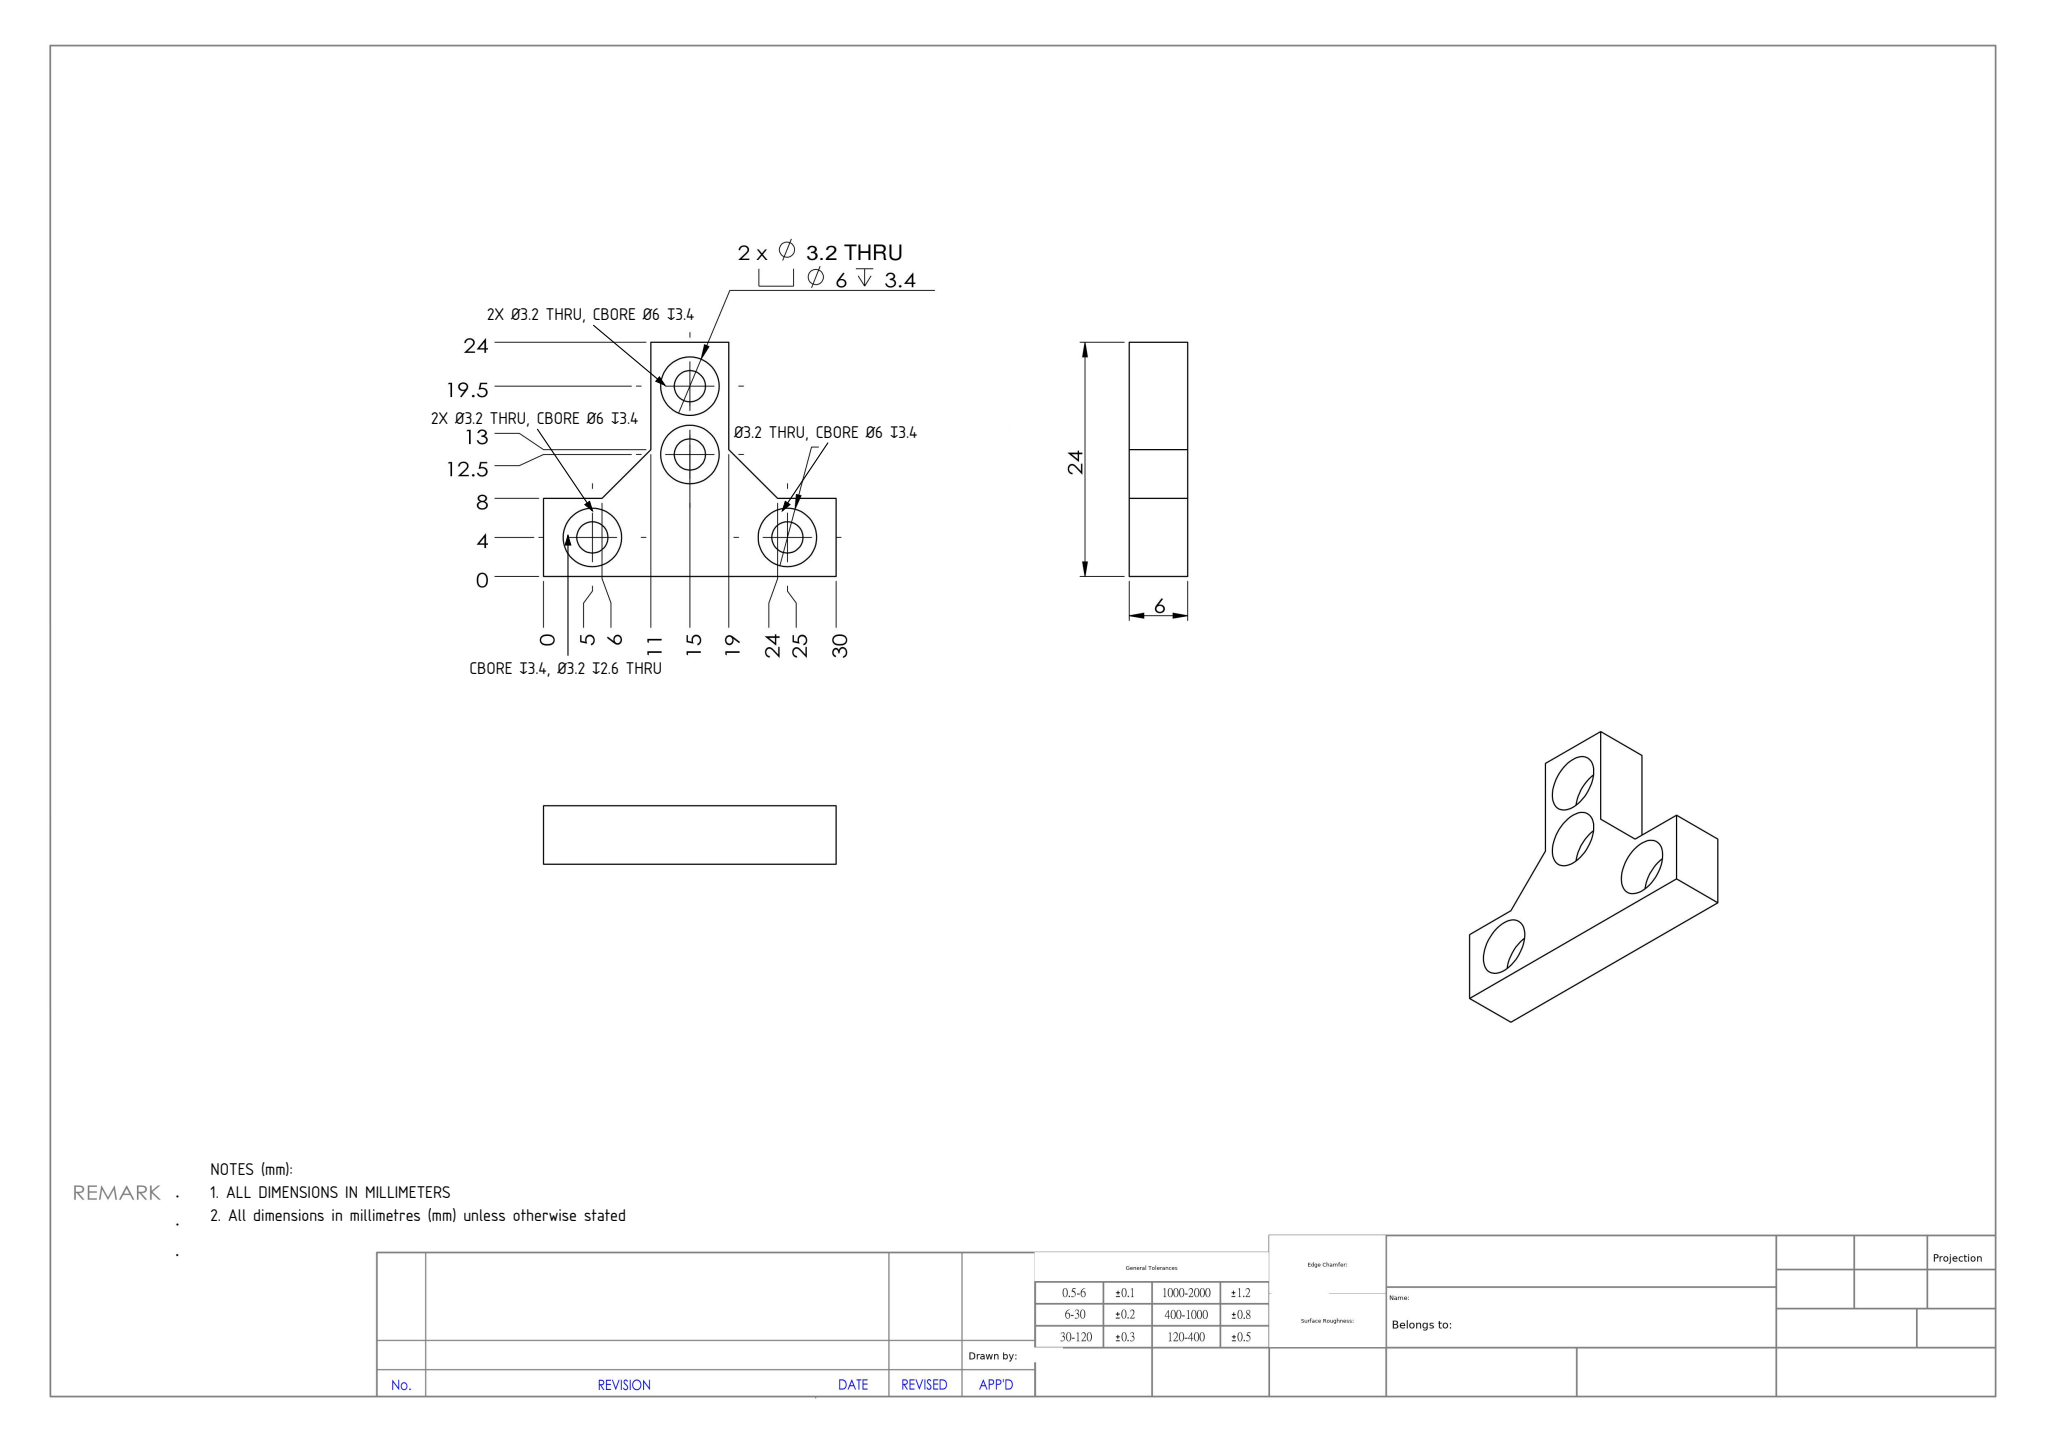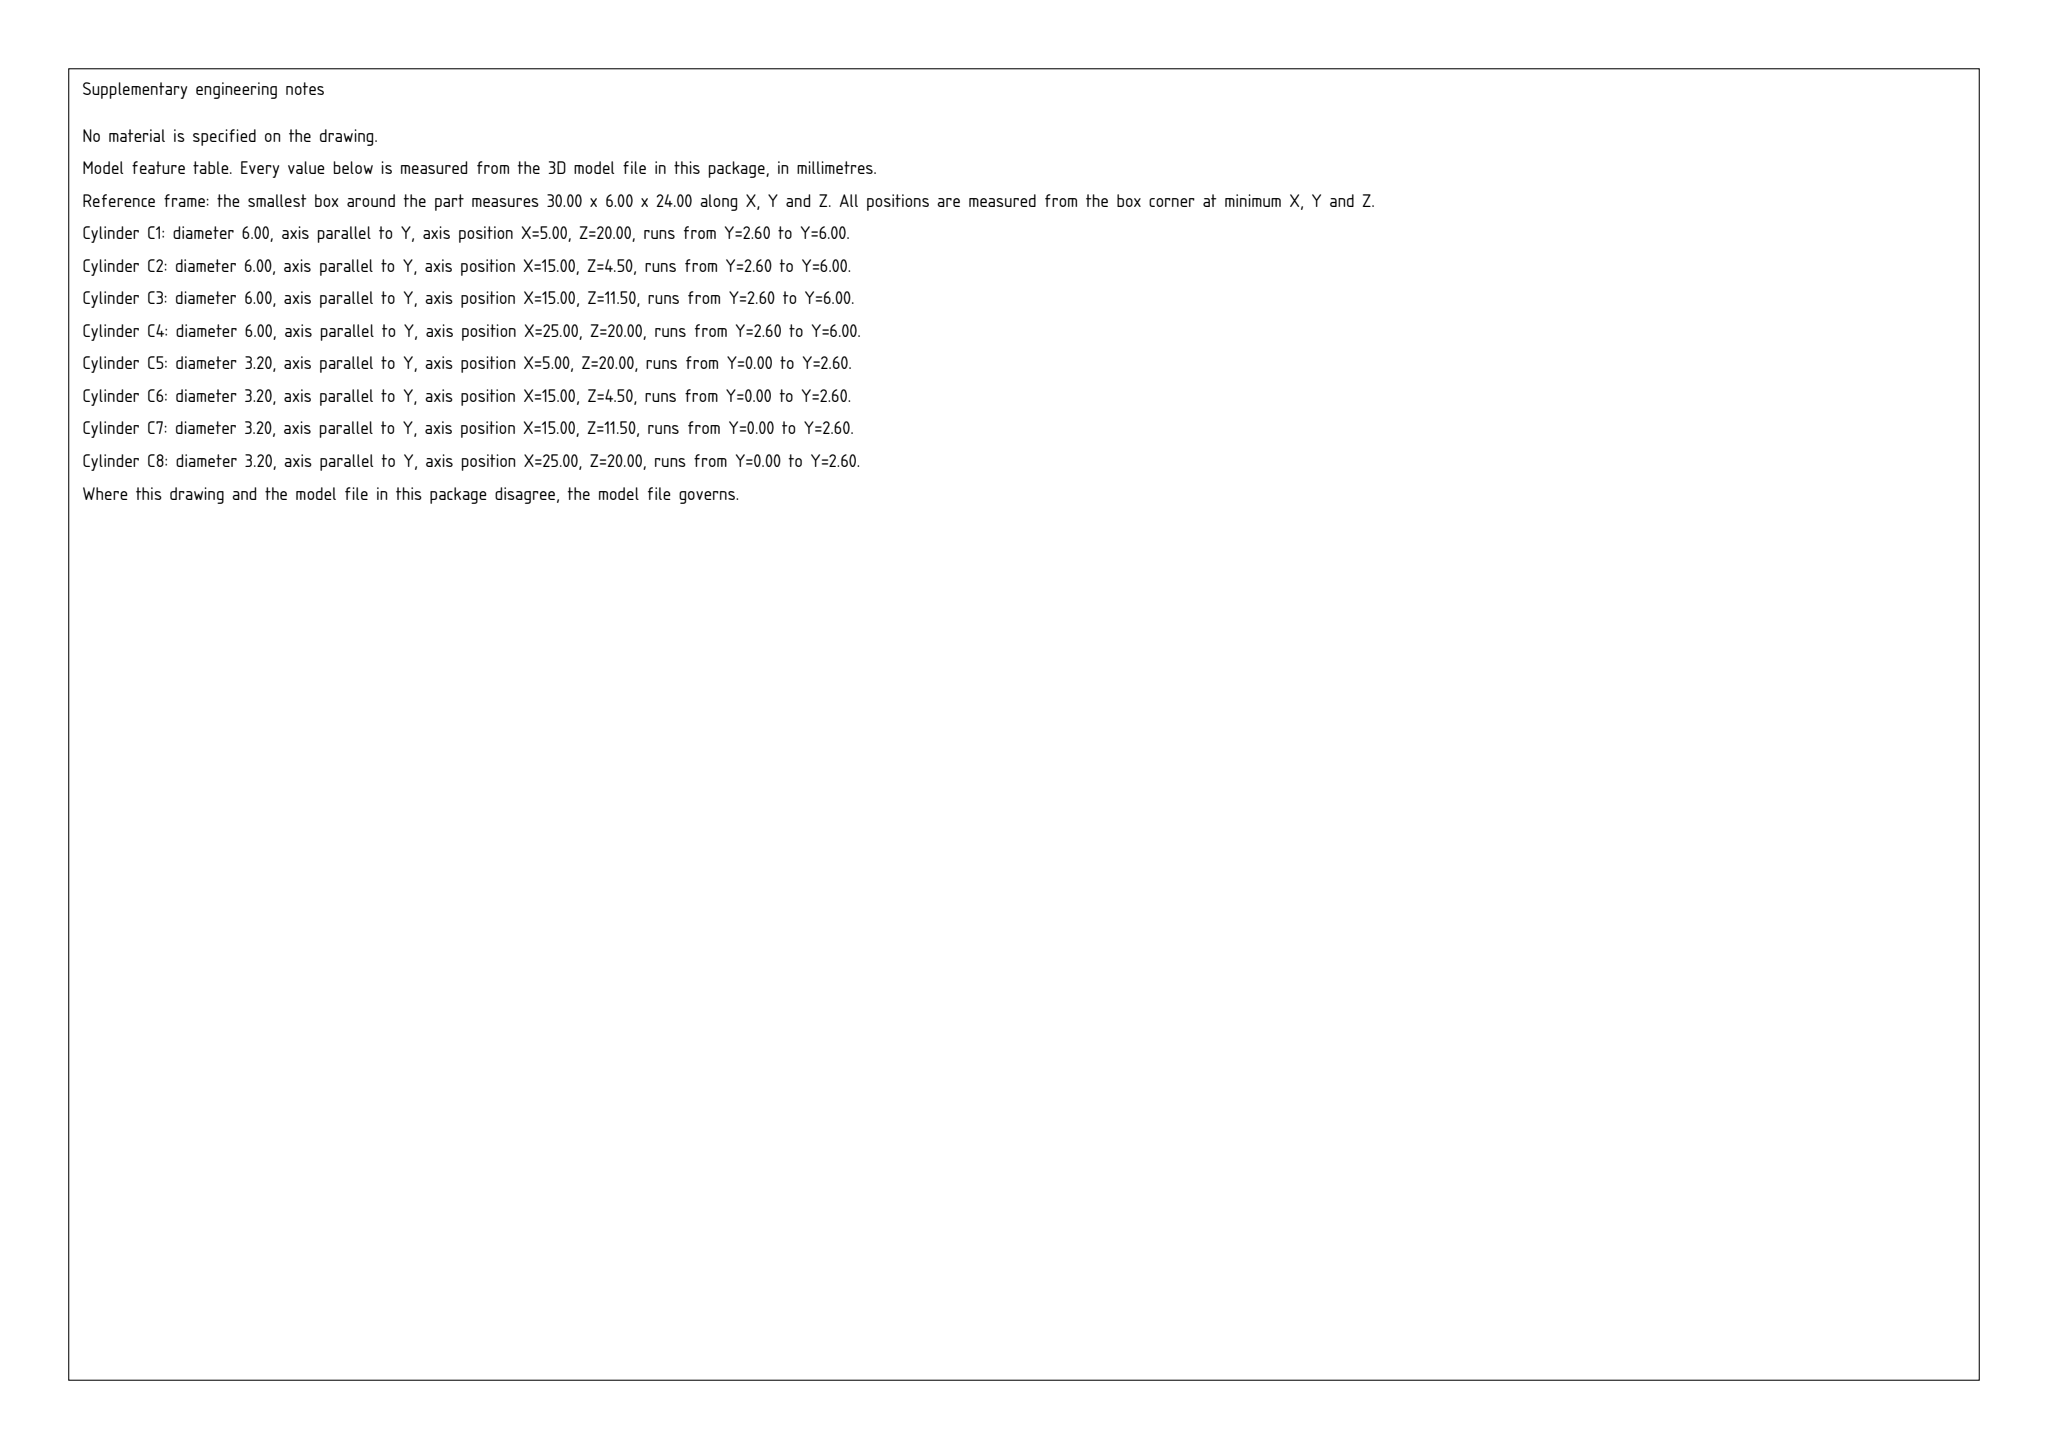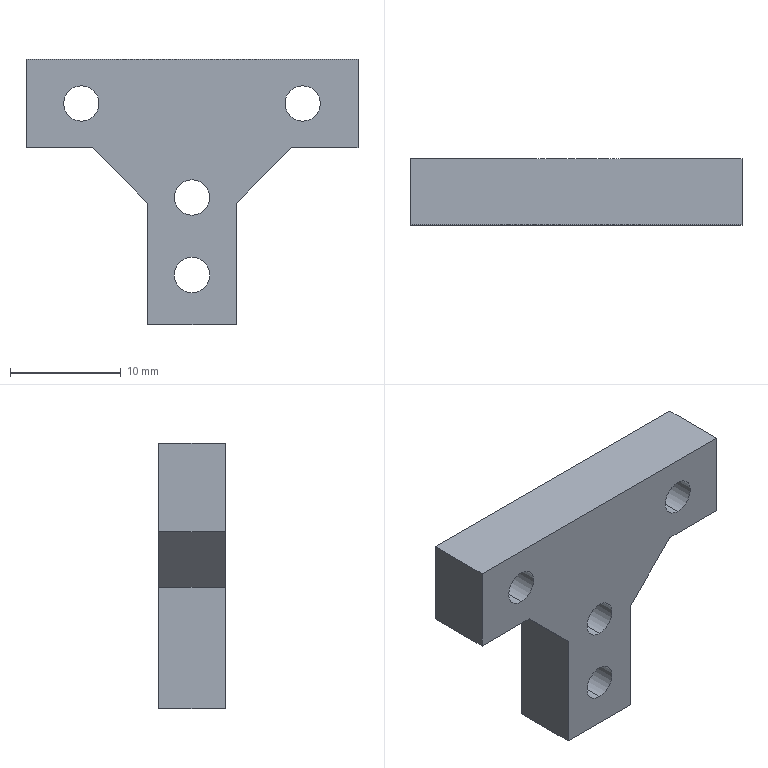Part | SolidWorks | mm | 1 solid | 32 faces | box 30 x 6 x 24 mm | volume 1890 mm3 | cylinder 16 | plane 16 | commonest cylinder face diameters 6 x8 3.2 x8
Drawing notes:
2X Ø3.2 THRU, CBORE Ø6 DP 3.4 (base holes) LOCATED AT X=5 AND X=25, Z=20 FROM BBOX MIN CORNER (4 FROM BASE BOTTOM EDGE) | from the solid: cylinders: [3.2,'y',[5,null,20],2.6] and [3.2,'y',[25,null,20],2.6]; [6.0,'y',[5,null,20],3.4] and [6.0,'y',[25,null,20],3.4]
ALL DIMENSIONS IN MILLIMETERS | from the solid: STEP model facts stated in mm (bbox_xyz 30.0 x 6.0 x 24.0 mm)
2X Ø3.2 THRU, C'BORE Ø6 DP 3.4 from front face (base holes), located X=5 and X=25, Z=20 from bbox min corner | from the solid: cylinders [3.2,'y',[5,null,20],2.6] and [3.2,'y',[25,null,20],2.6]; cylinders [6.0,'y',[5,null,20],3.4] and [6.0,'y',[25,null,20],3.4]
Counterbore depth 3.4 into 6 thick plate; hole Ø3.2 continues 2.6 THRU remaining wall | from the solid: axis_planes y=0, y=2.6, y=6.0 with cylinder lengths 3.4 (Ø6) + 2.6 (Ø3.2)
All dimensions in millimetres (mm) unless otherwise stated | from the solid: STEP model units: mm, bbox_xyz [30.0, 6.0, 24.0]
RIB HOLES: 2X Ø3.2 THRU, C'BORE Ø6 DP 3.4 FROM FRONT FACE (Y=6), ON AXIS X=15 FROM LEFT EDGE, AT Z=12.5 AND Z=19.5 ABOVE BASE BOTTOM EDGE (Z=0). TOTAL 4X Ø3.2 THRU, C'BORE Ø6 DP 3.4 ON PART. | from the solid: cylinders [3.2, y, [15,null,4.5], 2.6] and [3.2, y, [15,null,11.5], 2.6] with [6.0, y, [15,null,4.5], 3.4] and [6.0, y, [15,null,11.5], 3.4]; bbox_xyz 30x6x24 (Z from bottom = 24 - STEP z)
build123d program:
from build123d import *

# Parameters (mm, degrees)
SKETCH1_W                                         = 8
SKETCH1_H                                         = 16
BOSS_EXTRUDE1_DEPTH                               = 6
HOLE_SIZE_ACCORDING_TO_TYPE_1_FOR_HEX_D           = 3.2
HOLE_SIZE_ACCORDING_TO_TYPE_1_FOR_HEX_CBORE_D     = 6
HOLE_SIZE_ACCORDING_TO_TYPE_1_FOR_HEX_CBORE_DEPTH = 3.4
CHAMFER1_SIZE                                     = 5
HOLE_SIZE_ACCORDING_TO_TYPE_2_FOR_HEX_D           = 3.2
HOLE_SIZE_ACCORDING_TO_TYPE_2_FOR_HEX_CBORE_D     = 6
HOLE_SIZE_ACCORDING_TO_TYPE_2_FOR_HEX_CBORE_DEPTH = 3.4


with BuildPart() as part:
    # Sketch1 → Boss-Extrude1 (new body)
    with BuildSketch(Plane(origin=(0, 0, 0), x_dir=(1, 0, 0), z_dir=(0, 1, 0))):
        Rectangle(SKETCH1_W, SKETCH1_H)
        Polygon((4, -8), (-4, -8), (-15, -8), (-15, -16), (15, -16), (15, -8), align=None)
    extrude(amount=BOSS_EXTRUDE1_DEPTH)

    # Hole Size _ according to_ Type 1 for Hex (through all)
    with Locations(Plane(origin=(0, 6, 0), x_dir=(1, 0, 0), z_dir=(0, 1, 0))):
        with Locations((0, 3.5), (0, -3.5)):
            CounterBoreHole(HOLE_SIZE_ACCORDING_TO_TYPE_1_FOR_HEX_D / 2, HOLE_SIZE_ACCORDING_TO_TYPE_1_FOR_HEX_CBORE_D / 2, HOLE_SIZE_ACCORDING_TO_TYPE_1_FOR_HEX_CBORE_DEPTH)

    # Chamfer1
    chamfer1_edges = [part.edges().sort_by_distance(p)[0] for p in [
        (4, 3, 8),
        (-4, 3, 8),
    ]]
    chamfer(chamfer1_edges, length=CHAMFER1_SIZE)

    # Hole Size _ according to_ Type 2 for Hex (through all)
    with Locations(Plane(origin=(0, 6, 0), x_dir=(1, 0, 0), z_dir=(0, 1, 0))):
        with Locations((-10, -12), (10, -12)):
            CounterBoreHole(HOLE_SIZE_ACCORDING_TO_TYPE_2_FOR_HEX_D / 2, HOLE_SIZE_ACCORDING_TO_TYPE_2_FOR_HEX_CBORE_D / 2, HOLE_SIZE_ACCORDING_TO_TYPE_2_FOR_HEX_CBORE_DEPTH)


solid = part.part